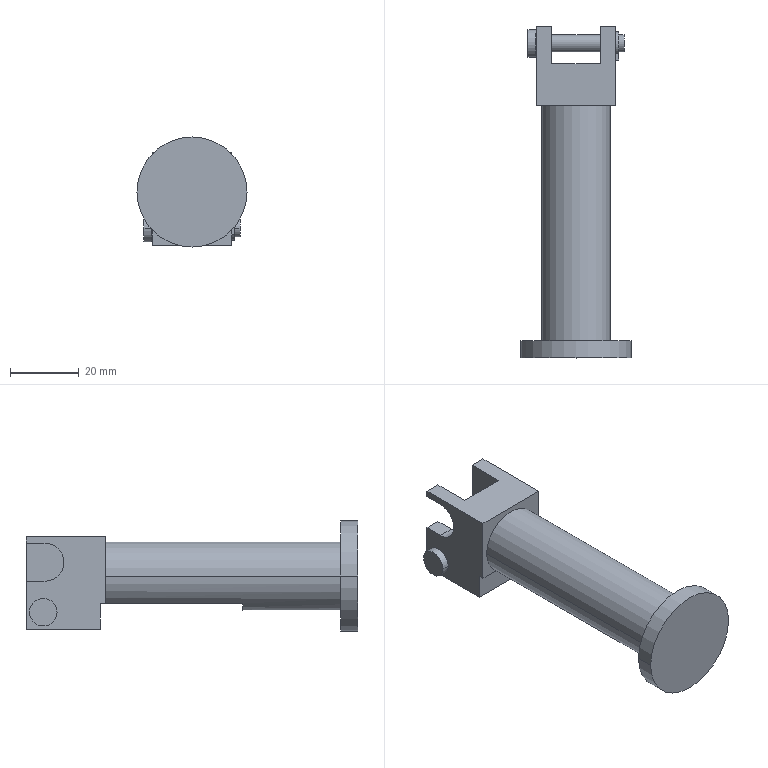Component | SolidWorks | RSDQA32-20DD-M9BL(0_0)-1_RSQ32-20D(0)_ROD-1 | 1 solid | 42 faces | volume 34696 mm3 | plane 26 | cylinder 16 | commonest cylinder face diameters 5 x6 20 x2 32 x2 11 x2 6.9 x2 8 x2